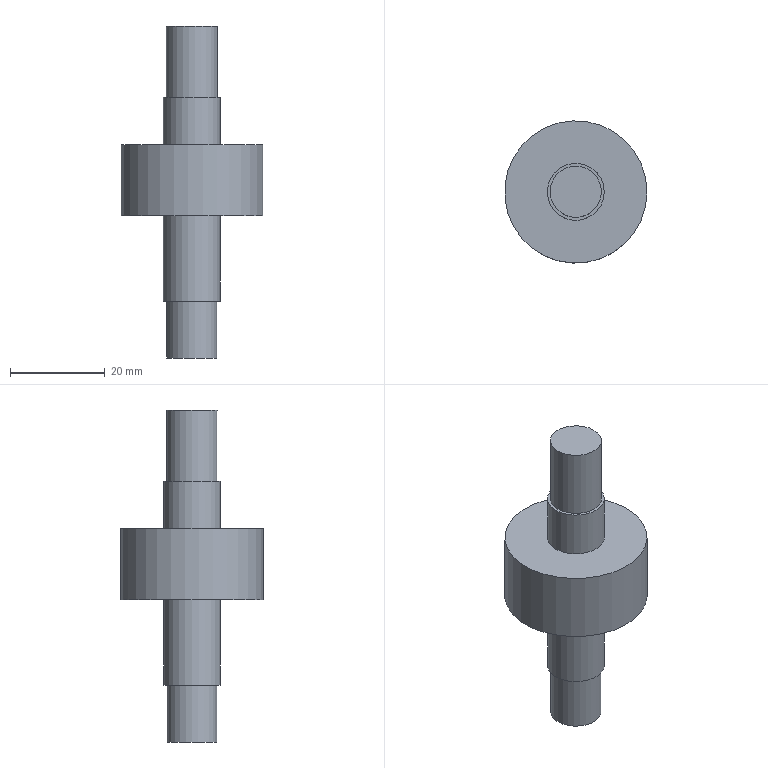Component | NX | MANDREL | 1 solid | 11 faces | box 30 x 30 x 70 mm | volume 16194 mm3 | plane 6 | cylinder 5 | commonest cylinder face diameters 12 x2 30 x1 10.579 x1 10.782 x1
STEP:
#1=CARTESIAN_POINT('',(0.,0.,0.));
#2=DIRECTION('',(0.,0.,1.));
#3=DIRECTION('',(1.,0.,0.));
#4=AXIS2_PLACEMENT_3D('',#1,#2,#3);
#5=CARTESIAN_POINT('',(6.,0.,18.));
#6=VERTEX_POINT('',#5);
#7=CARTESIAN_POINT('',(0.,0.,18.));
#8=DIRECTION('',(0.,0.,-1.));
#9=DIRECTION('',(1.,0.,0.));
#10=AXIS2_PLACEMENT_3D('',#7,#8,#9);
#11=CIRCLE('',#10,6.);
#12=CARTESIAN_POINT('',(0.,0.,43.));
#13=DIRECTION('',(0.,0.,-1.));
#14=DIRECTION('',(-1.,0.,0.));
#15=AXIS2_PLACEMENT_3D('',#12,#13,#14);
#16=CYLINDRICAL_SURFACE('',#15,6.);
#17=CARTESIAN_POINT('',(3.142,25.));
#18=DIRECTION('',(1.,0.));
#19=VECTOR('',#18,1.);
#20=LINE('',#17,#19);
#21=(GEOMETRIC_REPRESENTATION_CONTEXT(2)PARAMETRIC_REPRESENTATION_CONTEXT()REPRESENTATION_CONTEXT('',''));
#22=DEFINITIONAL_REPRESENTATION('',(#20),#21);
#23=PCURVE('',#16,#22);
#24=CARTESIAN_POINT('',(0.,0.,18.));
#25=DIRECTION('',(0.,0.,1.));
#26=DIRECTION('',(1.,0.,0.));
#27=AXIS2_PLACEMENT_3D('',#24,#25,#26);
#28=PLANE('',#27);
#29=CARTESIAN_POINT('',(6.,0.));
#30=CARTESIAN_POINT('',(6.,-10.392));
#31=CARTESIAN_POINT('',(-3.,-5.196));
#32=CARTESIAN_POINT('',(-12.,-0.));
#33=CARTESIAN_POINT('',(-3.,5.196));
#34=CARTESIAN_POINT('',(6.,10.392));
#35=CARTESIAN_POINT('',(6.,0.));
#36=(BOUNDED_CURVE()B_SPLINE_CURVE(2,(#29,#30,#31,#32,#33,#34,#35),.UNSPECIFIED.,.T.,.F.)B_SPLINE_CURVE_WITH_KNOTS((1,2,2,2,2,1),(-2.094,0.,2.094,4.189,6.283,8.378),.UNSPECIFIED.)CURVE()GEOMETRIC_REPRESENTATION_ITEM()RATIONAL_B_SPLINE_CURVE((1.,0.5,1.,0.5,1.,0.5,1.))REPRESENTATION_ITEM(''));
#37=(GEOMETRIC_REPRESENTATION_CONTEXT(2)PARAMETRIC_REPRESENTATION_CONTEXT()REPRESENTATION_CONTEXT('',''));
#38=DEFINITIONAL_REPRESENTATION('',(#36),#37);
#39=PCURVE('',#28,#38);
#40=SURFACE_CURVE('',#11,(#23,#39),.PCURVE_S1.);
#41=EDGE_CURVE('',#6,#6,#40,.T.);
#42=ORIENTED_EDGE('',*,*,#41,.F.);
#43=CARTESIAN_POINT('',(6.,0.,28.));
#44=VERTEX_POINT('',#43);
#45=CARTESIAN_POINT('',(6.,0.,28.));
#46=CARTESIAN_POINT('',(6.,0.,18.));
#47=B_SPLINE_CURVE_WITH_KNOTS('',1,(#45,#46),.UNSPECIFIED.,.F.,.F.,(2,2),(15.,25.),.PIECEWISE_BEZIER_KNOTS.);
#48=CARTESIAN_POINT('',(3.142,0.));
#49=DIRECTION('',(0.,1.));
#50=VECTOR('',#49,1.);
#51=LINE('',#48,#50);
#52=(GEOMETRIC_REPRESENTATION_CONTEXT(2)PARAMETRIC_REPRESENTATION_CONTEXT()REPRESENTATION_CONTEXT('',''));
#53=DEFINITIONAL_REPRESENTATION('',(#51),#52);
#54=PCURVE('',#16,#53);
#55=CARTESIAN_POINT('',(9.425,0.));
#56=DIRECTION('',(0.,1.));
#57=VECTOR('',#56,1.);
#58=LINE('',#55,#57);
#59=(GEOMETRIC_REPRESENTATION_CONTEXT(2)PARAMETRIC_REPRESENTATION_CONTEXT()REPRESENTATION_CONTEXT('',''));
#60=DEFINITIONAL_REPRESENTATION('',(#58),#59);
#61=PCURVE('',#16,#60);
#62=SEAM_CURVE('',#47,(#54,#61),.PCURVE_S1.);
#63=EDGE_CURVE('',#44,#6,#62,.T.);
#64=ORIENTED_EDGE('',*,*,#63,.F.);
#65=CARTESIAN_POINT('',(0.,0.,28.));
#66=DIRECTION('',(0.,0.,1.));
#67=DIRECTION('',(1.,0.,0.));
#68=AXIS2_PLACEMENT_3D('',#65,#66,#67);
#69=CIRCLE('',#68,6.);
#70=CARTESIAN_POINT('',(9.425,15.));
#71=DIRECTION('',(-1.,0.));
#72=VECTOR('',#71,1.);
#73=LINE('',#70,#72);
#74=(GEOMETRIC_REPRESENTATION_CONTEXT(2)PARAMETRIC_REPRESENTATION_CONTEXT()REPRESENTATION_CONTEXT('',''));
#75=DEFINITIONAL_REPRESENTATION('',(#73),#74);
#76=PCURVE('',#16,#75);
#77=CARTESIAN_POINT('',(0.,0.,28.));
#78=DIRECTION('',(0.,0.,1.));
#79=DIRECTION('',(1.,0.,0.));
#80=AXIS2_PLACEMENT_3D('',#77,#78,#79);
#81=PLANE('',#80);
#82=CARTESIAN_POINT('',(0.,0.));
#83=DIRECTION('',(1.,0.));
#84=AXIS2_PLACEMENT_2D('',#82,#83);
#85=CIRCLE('',#84,6.);
#86=(GEOMETRIC_REPRESENTATION_CONTEXT(2)PARAMETRIC_REPRESENTATION_CONTEXT()REPRESENTATION_CONTEXT('',''));
#87=DEFINITIONAL_REPRESENTATION('',(#85),#86);
#88=PCURVE('',#81,#87);
#89=SURFACE_CURVE('',#69,(#76,#88),.PCURVE_S1.);
#90=EDGE_CURVE('',#44,#44,#89,.T.);
#91=ORIENTED_EDGE('',*,*,#90,.F.);
#92=ORIENTED_EDGE('',*,*,#63,.T.);
#93=EDGE_LOOP('',(#42,#64,#91,#92));
#94=FACE_BOUND('',#93,.T.);
#95=ADVANCED_FACE('',(#94),#16,.T.);
#96=CARTESIAN_POINT('',(15.,0.,18.));
#97=VERTEX_POINT('',#96);
#98=CARTESIAN_POINT('',(0.,0.,18.));
#99=DIRECTION('',(0.,0.,1.));
#100=DIRECTION('',(1.,0.,0.));
#101=AXIS2_PLACEMENT_3D('',#98,#99,#100);
#102=CIRCLE('',#101,15.);
#103=CARTESIAN_POINT('',(0.,0.,18.));
#104=DIRECTION('',(0.,0.,-1.));
#105=DIRECTION('',(-1.,0.,0.));
#106=AXIS2_PLACEMENT_3D('',#103,#104,#105);
#107=CYLINDRICAL_SURFACE('',#106,15.);
#108=CARTESIAN_POINT('',(9.425,0.));
#109=DIRECTION('',(-1.,0.));
#110=VECTOR('',#109,1.);
#111=LINE('',#108,#110);
#112=(GEOMETRIC_REPRESENTATION_CONTEXT(2)PARAMETRIC_REPRESENTATION_CONTEXT()REPRESENTATION_CONTEXT('',''));
#113=DEFINITIONAL_REPRESENTATION('',(#111),#112);
#114=PCURVE('',#107,#113);
#115=CARTESIAN_POINT('',(0.,0.));
#116=DIRECTION('',(1.,0.));
#117=AXIS2_PLACEMENT_2D('',#115,#116);
#118=CIRCLE('',#117,15.);
#119=(GEOMETRIC_REPRESENTATION_CONTEXT(2)PARAMETRIC_REPRESENTATION_CONTEXT()REPRESENTATION_CONTEXT('',''));
#120=DEFINITIONAL_REPRESENTATION('',(#118),#119);
#121=PCURVE('',#28,#120);
#122=SURFACE_CURVE('',#102,(#114,#121),.PCURVE_S1.);
#123=EDGE_CURVE('',#97,#97,#122,.T.);
#124=ORIENTED_EDGE('',*,*,#123,.F.);
#125=CARTESIAN_POINT('',(15.,0.,3.));
#126=VERTEX_POINT('',#125);
#127=CARTESIAN_POINT('',(15.,0.,18.));
#128=CARTESIAN_POINT('',(15.,0.,3.));
#129=B_SPLINE_CURVE_WITH_KNOTS('',1,(#127,#128),.UNSPECIFIED.,.F.,.F.,(2,2),(0.,15.),.PIECEWISE_BEZIER_KNOTS.);
#130=CARTESIAN_POINT('',(9.425,0.));
#131=DIRECTION('',(0.,1.));
#132=VECTOR('',#131,1.);
#133=LINE('',#130,#132);
#134=(GEOMETRIC_REPRESENTATION_CONTEXT(2)PARAMETRIC_REPRESENTATION_CONTEXT()REPRESENTATION_CONTEXT('',''));
#135=DEFINITIONAL_REPRESENTATION('',(#133),#134);
#136=PCURVE('',#107,#135);
#137=CARTESIAN_POINT('',(3.142,0.));
#138=DIRECTION('',(0.,1.));
#139=VECTOR('',#138,1.);
#140=LINE('',#137,#139);
#141=(GEOMETRIC_REPRESENTATION_CONTEXT(2)PARAMETRIC_REPRESENTATION_CONTEXT()REPRESENTATION_CONTEXT('',''));
#142=DEFINITIONAL_REPRESENTATION('',(#140),#141);
#143=PCURVE('',#107,#142);
#144=SEAM_CURVE('',#129,(#136,#143),.PCURVE_S1.);
#145=EDGE_CURVE('',#97,#126,#144,.T.);
#146=ORIENTED_EDGE('',*,*,#145,.T.);
#147=CARTESIAN_POINT('',(0.,0.,3.));
#148=DIRECTION('',(0.,0.,1.));
#149=DIRECTION('',(1.,0.,0.));
#150=AXIS2_PLACEMENT_3D('',#147,#148,#149);
#151=CIRCLE('',#150,15.);
#152=CARTESIAN_POINT('',(9.425,15.));
#153=DIRECTION('',(-1.,0.));
#154=VECTOR('',#153,1.);
#155=LINE('',#152,#154);
#156=(GEOMETRIC_REPRESENTATION_CONTEXT(2)PARAMETRIC_REPRESENTATION_CONTEXT()REPRESENTATION_CONTEXT('',''));
#157=DEFINITIONAL_REPRESENTATION('',(#155),#156);
#158=PCURVE('',#107,#157);
#159=CARTESIAN_POINT('',(0.,0.,3.));
#160=DIRECTION('',(0.,0.,1.));
#161=DIRECTION('',(1.,0.,0.));
#162=AXIS2_PLACEMENT_3D('',#159,#160,#161);
#163=PLANE('',#162);
#164=CARTESIAN_POINT('',(0.,0.));
#165=DIRECTION('',(1.,0.));
#166=AXIS2_PLACEMENT_2D('',#164,#165);
#167=CIRCLE('',#166,15.);
#168=(GEOMETRIC_REPRESENTATION_CONTEXT(2)PARAMETRIC_REPRESENTATION_CONTEXT()REPRESENTATION_CONTEXT('',''));
#169=DEFINITIONAL_REPRESENTATION('',(#167),#168);
#170=PCURVE('',#163,#169);
#171=SURFACE_CURVE('',#151,(#158,#170),.PCURVE_S1.);
#172=EDGE_CURVE('',#126,#126,#171,.T.);
#173=ORIENTED_EDGE('',*,*,#172,.T.);
#174=ORIENTED_EDGE('',*,*,#145,.F.);
#175=EDGE_LOOP('',(#124,#146,#173,#174));
#176=FACE_BOUND('',#175,.T.);
#177=ADVANCED_FACE('',(#176),#107,.T.);
#178=ORIENTED_EDGE('',*,*,#41,.T.);
#179=EDGE_LOOP('',(#178));
#180=FACE_BOUND('',#179,.T.);
#181=ORIENTED_EDGE('',*,*,#123,.T.);
#182=EDGE_LOOP('',(#181));
#183=FACE_BOUND('',#182,.T.);
#184=ADVANCED_FACE('',(#180,#183),#28,.T.);
#185=CARTESIAN_POINT('',(6.,0.,3.));
#186=VERTEX_POINT('',#185);
#187=CARTESIAN_POINT('',(0.,0.,3.));
#188=DIRECTION('',(0.,0.,-1.));
#189=DIRECTION('',(1.,0.,0.));
#190=AXIS2_PLACEMENT_3D('',#187,#188,#189);
#191=CIRCLE('',#190,6.);
#192=CARTESIAN_POINT('',(6.,0.));
#193=CARTESIAN_POINT('',(6.,-10.392));
#194=CARTESIAN_POINT('',(-3.,-5.196));
#195=CARTESIAN_POINT('',(-12.,-0.));
#196=CARTESIAN_POINT('',(-3.,5.196));
#197=CARTESIAN_POINT('',(6.,10.392));
#198=CARTESIAN_POINT('',(6.,0.));
#199=(BOUNDED_CURVE()B_SPLINE_CURVE(2,(#192,#193,#194,#195,#196,#197,#198),.UNSPECIFIED.,.T.,.F.)B_SPLINE_CURVE_WITH_KNOTS((1,2,2,2,2,1),(-2.094,0.,2.094,4.189,6.283,8.378),.UNSPECIFIED.)CURVE()GEOMETRIC_REPRESENTATION_ITEM()RATIONAL_B_SPLINE_CURVE((1.,0.5,1.,0.5,1.,0.5,1.))REPRESENTATION_ITEM(''));
#200=(GEOMETRIC_REPRESENTATION_CONTEXT(2)PARAMETRIC_REPRESENTATION_CONTEXT()REPRESENTATION_CONTEXT('',''));
#201=DEFINITIONAL_REPRESENTATION('',(#199),#200);
#202=PCURVE('',#163,#201);
#203=CARTESIAN_POINT('',(0.,0.,43.));
#204=DIRECTION('',(0.,0.,-1.));
#205=DIRECTION('',(-1.,0.,0.));
#206=AXIS2_PLACEMENT_3D('',#203,#204,#205);
#207=CYLINDRICAL_SURFACE('',#206,6.);
#208=CARTESIAN_POINT('',(3.142,40.));
#209=DIRECTION('',(1.,0.));
#210=VECTOR('',#209,1.);
#211=LINE('',#208,#210);
#212=(GEOMETRIC_REPRESENTATION_CONTEXT(2)PARAMETRIC_REPRESENTATION_CONTEXT()REPRESENTATION_CONTEXT('',''));
#213=DEFINITIONAL_REPRESENTATION('',(#211),#212);
#214=PCURVE('',#207,#213);
#215=SURFACE_CURVE('',#191,(#202,#214),.PCURVE_S1.);
#216=EDGE_CURVE('',#186,#186,#215,.T.);
#217=ORIENTED_EDGE('',*,*,#216,.F.);
#218=EDGE_LOOP('',(#217));
#219=FACE_BOUND('',#218,.T.);
#220=ORIENTED_EDGE('',*,*,#172,.F.);
#221=EDGE_LOOP('',(#220));
#222=FACE_BOUND('',#221,.T.);
#223=ADVANCED_FACE('',(#219,#222),#163,.F.);
#224=CARTESIAN_POINT('',(6.,0.,-15.));
#225=VERTEX_POINT('',#224);
#226=CARTESIAN_POINT('',(0.,0.,-15.));
#227=DIRECTION('',(0.,0.,1.));
#228=DIRECTION('',(1.,0.,0.));
#229=AXIS2_PLACEMENT_3D('',#226,#227,#228);
#230=CIRCLE('',#229,6.);
#231=CARTESIAN_POINT('',(9.425,58.));
#232=DIRECTION('',(-1.,0.));
#233=VECTOR('',#232,1.);
#234=LINE('',#231,#233);
#235=(GEOMETRIC_REPRESENTATION_CONTEXT(2)PARAMETRIC_REPRESENTATION_CONTEXT()REPRESENTATION_CONTEXT('',''));
#236=DEFINITIONAL_REPRESENTATION('',(#234),#235);
#237=PCURVE('',#207,#236);
#238=CARTESIAN_POINT('',(0.,0.,-15.));
#239=DIRECTION('',(0.,0.,1.));
#240=DIRECTION('',(1.,0.,0.));
#241=AXIS2_PLACEMENT_3D('',#238,#239,#240);
#242=PLANE('',#241);
#243=CARTESIAN_POINT('',(0.,0.));
#244=DIRECTION('',(1.,0.));
#245=AXIS2_PLACEMENT_2D('',#243,#244);
#246=CIRCLE('',#245,6.);
#247=(GEOMETRIC_REPRESENTATION_CONTEXT(2)PARAMETRIC_REPRESENTATION_CONTEXT()REPRESENTATION_CONTEXT('',''));
#248=DEFINITIONAL_REPRESENTATION('',(#246),#247);
#249=PCURVE('',#242,#248);
#250=SURFACE_CURVE('',#230,(#237,#249),.PCURVE_S1.);
#251=EDGE_CURVE('',#225,#225,#250,.T.);
#252=ORIENTED_EDGE('',*,*,#251,.T.);
#253=CARTESIAN_POINT('',(6.,0.,3.));
#254=CARTESIAN_POINT('',(6.,0.,-15.));
#255=B_SPLINE_CURVE_WITH_KNOTS('',1,(#253,#254),.UNSPECIFIED.,.F.,.F.,(2,2),(40.,58.),.PIECEWISE_BEZIER_KNOTS.);
#256=CARTESIAN_POINT('',(3.142,0.));
#257=DIRECTION('',(0.,1.));
#258=VECTOR('',#257,1.);
#259=LINE('',#256,#258);
#260=(GEOMETRIC_REPRESENTATION_CONTEXT(2)PARAMETRIC_REPRESENTATION_CONTEXT()REPRESENTATION_CONTEXT('',''));
#261=DEFINITIONAL_REPRESENTATION('',(#259),#260);
#262=PCURVE('',#207,#261);
#263=CARTESIAN_POINT('',(9.425,0.));
#264=DIRECTION('',(0.,1.));
#265=VECTOR('',#264,1.);
#266=LINE('',#263,#265);
#267=(GEOMETRIC_REPRESENTATION_CONTEXT(2)PARAMETRIC_REPRESENTATION_CONTEXT()REPRESENTATION_CONTEXT('',''));
#268=DEFINITIONAL_REPRESENTATION('',(#266),#267);
#269=PCURVE('',#207,#268);
#270=SEAM_CURVE('',#255,(#262,#269),.PCURVE_S1.);
#271=EDGE_CURVE('',#186,#225,#270,.T.);
#272=ORIENTED_EDGE('',*,*,#271,.F.);
#273=ORIENTED_EDGE('',*,*,#216,.T.);
#274=ORIENTED_EDGE('',*,*,#271,.T.);
#275=EDGE_LOOP('',(#252,#272,#273,#274));
#276=FACE_BOUND('',#275,.T.);
#277=ADVANCED_FACE('',(#276),#207,.T.);
#278=CARTESIAN_POINT('',(5.29,0.,-15.));
#279=VERTEX_POINT('',#278);
#280=CARTESIAN_POINT('',(0.,0.,-15.));
#281=DIRECTION('',(0.,0.,-1.));
#282=DIRECTION('',(1.,0.,0.));
#283=AXIS2_PLACEMENT_3D('',#280,#281,#282);
#284=CIRCLE('',#283,5.29);
#285=CARTESIAN_POINT('',(0.,0.,-15.));
#286=DIRECTION('',(0.,0.,-1.));
#287=DIRECTION('',(-1.,0.,0.));
#288=AXIS2_PLACEMENT_3D('',#285,#286,#287);
#289=CYLINDRICAL_SURFACE('',#288,5.29);
#290=CARTESIAN_POINT('',(3.142,0.));
#291=DIRECTION('',(1.,0.));
#292=VECTOR('',#291,1.);
#293=LINE('',#290,#292);
#294=(GEOMETRIC_REPRESENTATION_CONTEXT(2)PARAMETRIC_REPRESENTATION_CONTEXT()REPRESENTATION_CONTEXT('',''));
#295=DEFINITIONAL_REPRESENTATION('',(#293),#294);
#296=PCURVE('',#289,#295);
#297=CARTESIAN_POINT('',(5.29,0.));
#298=CARTESIAN_POINT('',(5.29,-9.162));
#299=CARTESIAN_POINT('',(-2.645,-4.581));
#300=CARTESIAN_POINT('',(-10.579,-0.));
#301=CARTESIAN_POINT('',(-2.645,4.581));
#302=CARTESIAN_POINT('',(5.29,9.162));
#303=CARTESIAN_POINT('',(5.29,0.));
#304=(BOUNDED_CURVE()B_SPLINE_CURVE(2,(#297,#298,#299,#300,#301,#302,#303),.UNSPECIFIED.,.T.,.F.)B_SPLINE_CURVE_WITH_KNOTS((1,2,2,2,2,1),(-2.094,0.,2.094,4.189,6.283,8.378),.UNSPECIFIED.)CURVE()GEOMETRIC_REPRESENTATION_ITEM()RATIONAL_B_SPLINE_CURVE((1.,0.5,1.,0.5,1.,0.5,1.))REPRESENTATION_ITEM(''));
#305=(GEOMETRIC_REPRESENTATION_CONTEXT(2)PARAMETRIC_REPRESENTATION_CONTEXT()REPRESENTATION_CONTEXT('',''));
#306=DEFINITIONAL_REPRESENTATION('',(#304),#305);
#307=PCURVE('',#242,#306);
#308=SURFACE_CURVE('',#284,(#296,#307),.PCURVE_S1.);
#309=EDGE_CURVE('',#279,#279,#308,.T.);
#310=ORIENTED_EDGE('',*,*,#309,.T.);
#311=CARTESIAN_POINT('',(5.29,0.,-27.));
#312=VERTEX_POINT('',#311);
#313=CARTESIAN_POINT('',(5.29,0.,-15.));
#314=CARTESIAN_POINT('',(5.29,0.,-27.));
#315=B_SPLINE_CURVE_WITH_KNOTS('',1,(#313,#314),.UNSPECIFIED.,.F.,.F.,(2,2),(0.,12.),.PIECEWISE_BEZIER_KNOTS.);
#316=CARTESIAN_POINT('',(9.425,0.));
#317=DIRECTION('',(0.,1.));
#318=VECTOR('',#317,1.);
#319=LINE('',#316,#318);
#320=(GEOMETRIC_REPRESENTATION_CONTEXT(2)PARAMETRIC_REPRESENTATION_CONTEXT()REPRESENTATION_CONTEXT('',''));
#321=DEFINITIONAL_REPRESENTATION('',(#319),#320);
#322=PCURVE('',#289,#321);
#323=CARTESIAN_POINT('',(3.142,0.));
#324=DIRECTION('',(0.,1.));
#325=VECTOR('',#324,1.);
#326=LINE('',#323,#325);
#327=(GEOMETRIC_REPRESENTATION_CONTEXT(2)PARAMETRIC_REPRESENTATION_CONTEXT()REPRESENTATION_CONTEXT('',''));
#328=DEFINITIONAL_REPRESENTATION('',(#326),#327);
#329=PCURVE('',#289,#328);
#330=SEAM_CURVE('',#315,(#322,#329),.PCURVE_S1.);
#331=EDGE_CURVE('',#279,#312,#330,.T.);
#332=ORIENTED_EDGE('',*,*,#331,.T.);
#333=CARTESIAN_POINT('',(0.,0.,-27.));
#334=DIRECTION('',(0.,0.,-1.));
#335=DIRECTION('',(1.,0.,0.));
#336=AXIS2_PLACEMENT_3D('',#333,#334,#335);
#337=CIRCLE('',#336,5.29);
#338=CARTESIAN_POINT('',(3.142,12.));
#339=DIRECTION('',(1.,0.));
#340=VECTOR('',#339,1.);
#341=LINE('',#338,#340);
#342=(GEOMETRIC_REPRESENTATION_CONTEXT(2)PARAMETRIC_REPRESENTATION_CONTEXT()REPRESENTATION_CONTEXT('',''));
#343=DEFINITIONAL_REPRESENTATION('',(#341),#342);
#344=PCURVE('',#289,#343);
#345=CARTESIAN_POINT('',(0.,0.,-27.));
#346=DIRECTION('',(0.,0.,1.));
#347=DIRECTION('',(1.,0.,0.));
#348=AXIS2_PLACEMENT_3D('',#345,#346,#347);
#349=PLANE('',#348);
#350=CARTESIAN_POINT('',(5.29,0.));
#351=CARTESIAN_POINT('',(5.29,-9.162));
#352=CARTESIAN_POINT('',(-2.645,-4.581));
#353=CARTESIAN_POINT('',(-10.579,-0.));
#354=CARTESIAN_POINT('',(-2.645,4.581));
#355=CARTESIAN_POINT('',(5.29,9.162));
#356=CARTESIAN_POINT('',(5.29,0.));
#357=(BOUNDED_CURVE()B_SPLINE_CURVE(2,(#350,#351,#352,#353,#354,#355,#356),.UNSPECIFIED.,.T.,.F.)B_SPLINE_CURVE_WITH_KNOTS((1,2,2,2,2,1),(-2.094,0.,2.094,4.189,6.283,8.378),.UNSPECIFIED.)CURVE()GEOMETRIC_REPRESENTATION_ITEM()RATIONAL_B_SPLINE_CURVE((1.,0.5,1.,0.5,1.,0.5,1.))REPRESENTATION_ITEM(''));
#358=(GEOMETRIC_REPRESENTATION_CONTEXT(2)PARAMETRIC_REPRESENTATION_CONTEXT()REPRESENTATION_CONTEXT('',''));
#359=DEFINITIONAL_REPRESENTATION('',(#357),#358);
#360=PCURVE('',#349,#359);
#361=SURFACE_CURVE('',#337,(#344,#360),.PCURVE_S1.);
#362=EDGE_CURVE('',#312,#312,#361,.T.);
#363=ORIENTED_EDGE('',*,*,#362,.F.);
#364=ORIENTED_EDGE('',*,*,#331,.F.);
#365=EDGE_LOOP('',(#310,#332,#363,#364));
#366=FACE_BOUND('',#365,.T.);
#367=ADVANCED_FACE('',(#366),#289,.T.);
#368=ORIENTED_EDGE('',*,*,#309,.F.);
#369=EDGE_LOOP('',(#368));
#370=FACE_BOUND('',#369,.T.);
#371=ORIENTED_EDGE('',*,*,#251,.F.);
#372=EDGE_LOOP('',(#371));
#373=FACE_BOUND('',#372,.T.);
#374=ADVANCED_FACE('',(#370,#373),#242,.F.);
#375=ORIENTED_EDGE('',*,*,#362,.T.);
#376=EDGE_LOOP('',(#375));
#377=FACE_BOUND('',#376,.T.);
#378=ADVANCED_FACE('',(#377),#349,.F.);
#379=CARTESIAN_POINT('',(5.391,0.,28.));
#380=VERTEX_POINT('',#379);
#381=CARTESIAN_POINT('',(0.,0.,28.));
#382=DIRECTION('',(0.,0.,-1.));
#383=DIRECTION('',(1.,0.,0.));
#384=AXIS2_PLACEMENT_3D('',#381,#382,#383);
#385=CIRCLE('',#384,5.391);
#386=CARTESIAN_POINT('',(5.391,0.));
#387=CARTESIAN_POINT('',(5.391,-9.338));
#388=CARTESIAN_POINT('',(-2.696,-4.669));
#389=CARTESIAN_POINT('',(-10.782,-0.));
#390=CARTESIAN_POINT('',(-2.696,4.669));
#391=CARTESIAN_POINT('',(5.391,9.338));
#392=CARTESIAN_POINT('',(5.391,0.));
#393=(BOUNDED_CURVE()B_SPLINE_CURVE(2,(#386,#387,#388,#389,#390,#391,#392),.UNSPECIFIED.,.T.,.F.)B_SPLINE_CURVE_WITH_KNOTS((1,2,2,2,2,1),(-2.094,0.,2.094,4.189,6.283,8.378),.UNSPECIFIED.)CURVE()GEOMETRIC_REPRESENTATION_ITEM()RATIONAL_B_SPLINE_CURVE((1.,0.5,1.,0.5,1.,0.5,1.))REPRESENTATION_ITEM(''));
#394=(GEOMETRIC_REPRESENTATION_CONTEXT(2)PARAMETRIC_REPRESENTATION_CONTEXT()REPRESENTATION_CONTEXT('',''));
#395=DEFINITIONAL_REPRESENTATION('',(#393),#394);
#396=PCURVE('',#81,#395);
#397=CARTESIAN_POINT('',(0.,0.,44.));
#398=DIRECTION('',(0.,0.,-1.));
#399=DIRECTION('',(-1.,0.,0.));
#400=AXIS2_PLACEMENT_3D('',#397,#398,#399);
#401=CYLINDRICAL_SURFACE('',#400,5.391);
#402=CARTESIAN_POINT('',(3.142,16.));
#403=DIRECTION('',(1.,0.));
#404=VECTOR('',#403,1.);
#405=LINE('',#402,#404);
#406=(GEOMETRIC_REPRESENTATION_CONTEXT(2)PARAMETRIC_REPRESENTATION_CONTEXT()REPRESENTATION_CONTEXT('',''));
#407=DEFINITIONAL_REPRESENTATION('',(#405),#406);
#408=PCURVE('',#401,#407);
#409=SURFACE_CURVE('',#385,(#396,#408),.PCURVE_S1.);
#410=EDGE_CURVE('',#380,#380,#409,.T.);
#411=ORIENTED_EDGE('',*,*,#410,.T.);
#412=EDGE_LOOP('',(#411));
#413=FACE_BOUND('',#412,.T.);
#414=ORIENTED_EDGE('',*,*,#90,.T.);
#415=EDGE_LOOP('',(#414));
#416=FACE_BOUND('',#415,.T.);
#417=ADVANCED_FACE('',(#413,#416),#81,.T.);
#418=CARTESIAN_POINT('',(5.391,0.,43.));
#419=VERTEX_POINT('',#418);
#420=CARTESIAN_POINT('',(0.,0.,43.));
#421=DIRECTION('',(0.,0.,-1.));
#422=DIRECTION('',(1.,0.,0.));
#423=AXIS2_PLACEMENT_3D('',#420,#421,#422);
#424=CIRCLE('',#423,5.391);
#425=CARTESIAN_POINT('',(3.142,1.));
#426=DIRECTION('',(1.,0.));
#427=VECTOR('',#426,1.);
#428=LINE('',#425,#427);
#429=(GEOMETRIC_REPRESENTATION_CONTEXT(2)PARAMETRIC_REPRESENTATION_CONTEXT()REPRESENTATION_CONTEXT('',''));
#430=DEFINITIONAL_REPRESENTATION('',(#428),#429);
#431=PCURVE('',#401,#430);
#432=CARTESIAN_POINT('',(0.,0.,43.));
#433=DIRECTION('',(0.,0.,1.));
#434=DIRECTION('',(1.,0.,0.));
#435=AXIS2_PLACEMENT_3D('',#432,#433,#434);
#436=PLANE('',#435);
#437=CARTESIAN_POINT('',(5.391,0.));
#438=CARTESIAN_POINT('',(5.391,-9.338));
#439=CARTESIAN_POINT('',(-2.696,-4.669));
#440=CARTESIAN_POINT('',(-10.782,-0.));
#441=CARTESIAN_POINT('',(-2.696,4.669));
#442=CARTESIAN_POINT('',(5.391,9.338));
#443=CARTESIAN_POINT('',(5.391,0.));
#444=(BOUNDED_CURVE()B_SPLINE_CURVE(2,(#437,#438,#439,#440,#441,#442,#443),.UNSPECIFIED.,.T.,.F.)B_SPLINE_CURVE_WITH_KNOTS((1,2,2,2,2,1),(-2.094,0.,2.094,4.189,6.283,8.378),.UNSPECIFIED.)CURVE()GEOMETRIC_REPRESENTATION_ITEM()RATIONAL_B_SPLINE_CURVE((1.,0.5,1.,0.5,1.,0.5,1.))REPRESENTATION_ITEM(''));
#445=(GEOMETRIC_REPRESENTATION_CONTEXT(2)PARAMETRIC_REPRESENTATION_CONTEXT()REPRESENTATION_CONTEXT('',''));
#446=DEFINITIONAL_REPRESENTATION('',(#444),#445);
#447=PCURVE('',#436,#446);
#448=SURFACE_CURVE('',#424,(#431,#447),.PCURVE_S1.);
#449=EDGE_CURVE('',#419,#419,#448,.T.);
#450=ORIENTED_EDGE('',*,*,#449,.T.);
#451=CARTESIAN_POINT('',(5.391,0.,43.));
#452=CARTESIAN_POINT('',(5.391,0.,28.));
#453=B_SPLINE_CURVE_WITH_KNOTS('',1,(#451,#452),.UNSPECIFIED.,.F.,.F.,(2,2),(1.,16.),.PIECEWISE_BEZIER_KNOTS.);
#454=CARTESIAN_POINT('',(9.425,0.));
#455=DIRECTION('',(0.,1.));
#456=VECTOR('',#455,1.);
#457=LINE('',#454,#456);
#458=(GEOMETRIC_REPRESENTATION_CONTEXT(2)PARAMETRIC_REPRESENTATION_CONTEXT()REPRESENTATION_CONTEXT('',''));
#459=DEFINITIONAL_REPRESENTATION('',(#457),#458);
#460=PCURVE('',#401,#459);
#461=CARTESIAN_POINT('',(3.142,0.));
#462=DIRECTION('',(0.,1.));
#463=VECTOR('',#462,1.);
#464=LINE('',#461,#463);
#465=(GEOMETRIC_REPRESENTATION_CONTEXT(2)PARAMETRIC_REPRESENTATION_CONTEXT()REPRESENTATION_CONTEXT('',''));
#466=DEFINITIONAL_REPRESENTATION('',(#464),#465);
#467=PCURVE('',#401,#466);
#468=SEAM_CURVE('',#453,(#460,#467),.PCURVE_S1.);
#469=EDGE_CURVE('',#419,#380,#468,.T.);
#470=ORIENTED_EDGE('',*,*,#469,.T.);
#471=ORIENTED_EDGE('',*,*,#410,.F.);
#472=ORIENTED_EDGE('',*,*,#469,.F.);
#473=EDGE_LOOP('',(#450,#470,#471,#472));
#474=FACE_BOUND('',#473,.T.);
#475=ADVANCED_FACE('',(#474),#401,.T.);
#476=ORIENTED_EDGE('',*,*,#449,.F.);
#477=EDGE_LOOP('',(#476));
#478=FACE_BOUND('',#477,.T.);
#479=ADVANCED_FACE('',(#478),#436,.T.);
#480=CLOSED_SHELL('',(#95,#177,#184,#223,#277,#367,#374,#378,#417,#475,#479));
#481=MANIFOLD_SOLID_BREP('',#480);
#482=(LENGTH_UNIT()NAMED_UNIT(*)SI_UNIT(.MILLI.,.METRE.));
#483=UNCERTAINTY_MEASURE_WITH_UNIT(LENGTH_MEASURE(0.00001),#482,'','');
#484=(NAMED_UNIT(*)PLANE_ANGLE_UNIT()SI_UNIT($,.RADIAN.));
#485=(NAMED_UNIT(*)SI_UNIT($,.STERADIAN.)SOLID_ANGLE_UNIT());
#486=(GEOMETRIC_REPRESENTATION_CONTEXT(3)GLOBAL_UNCERTAINTY_ASSIGNED_CONTEXT((#483))GLOBAL_UNIT_ASSIGNED_CONTEXT((#482,#484,#485))REPRESENTATION_CONTEXT('',''));
#487=ADVANCED_BREP_SHAPE_REPRESENTATION('',(#4,#481),#486);